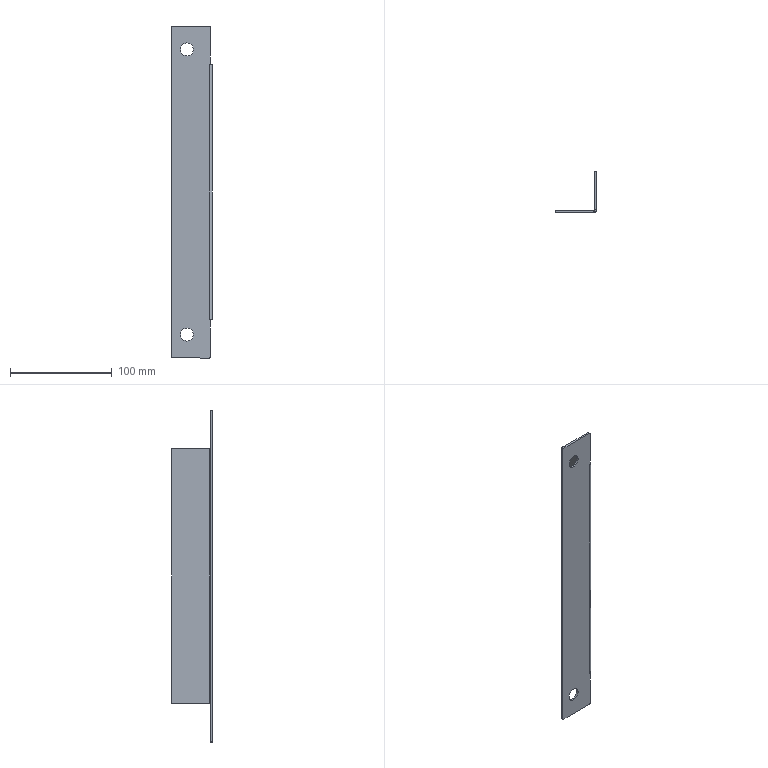Component | SolidWorks | BaseBracketAssembly-1_BaseBracketDepth-9 | 1 solid | 30 faces | box 40 x 40 x 326 mm | volume 43936 mm3 | plane 24 | cylinder 6 | commonest cylinder face diameters 12.639 x4 1 x1 5 x1 | material 2.0mm Cold Rolled Plate
STEP:
#1=COLOUR_RGB('',0.7922,0.8196,0.9333);
#2=FILL_AREA_STYLE_COLOUR('',#1);
#3=FILL_AREA_STYLE('',(#2));
#4=SURFACE_STYLE_FILL_AREA(#3);
#5=SURFACE_SIDE_STYLE('',(#4));
#6=SURFACE_STYLE_USAGE(.BOTH.,#5);
#7=PRESENTATION_STYLE_ASSIGNMENT((#6));
#8=CARTESIAN_POINT('',(9.08,-50.005,25.933));
#9=VERTEX_POINT('',#8);
#10=CARTESIAN_POINT('',(9.08,-50.005,25.436));
#11=VERTEX_POINT('',#10);
#12=CARTESIAN_POINT('',(9.08,-50.005,25.685));
#13=DIRECTION('',(-0.,1.,0.));
#14=DIRECTION('',(-0.,0.,-1.));
#15=AXIS2_PLACEMENT_3D('',#12,#13,#14);
#16=CIRCLE('',#15,0.2488);
#17=EDGE_CURVE('',#9,#11,#16,.T.);
#18=ORIENTED_EDGE('',*,*,#17,.F.);
#19=CARTESIAN_POINT('',(9.08,-49.926,25.933));
#20=VERTEX_POINT('',#19);
#21=CARTESIAN_POINT('',(9.08,-50.32,25.933));
#22=DIRECTION('',(-0.,1.,0.));
#23=VECTOR('',#22,39.37);
#24=LINE('',#21,#23);
#25=EDGE_CURVE('',#9,#20,#24,.T.);
#26=ORIENTED_EDGE('',*,*,#25,.T.);
#27=CARTESIAN_POINT('',(9.08,-49.926,25.436));
#28=VERTEX_POINT('',#27);
#29=CARTESIAN_POINT('',(9.08,-49.926,25.685));
#30=DIRECTION('',(-0.,1.,0.));
#31=DIRECTION('',(-0.,0.,-1.));
#32=AXIS2_PLACEMENT_3D('',#29,#30,#31);
#33=CIRCLE('',#32,0.2488);
#34=EDGE_CURVE('',#20,#28,#33,.T.);
#35=ORIENTED_EDGE('',*,*,#34,.T.);
#36=CARTESIAN_POINT('',(9.08,-50.32,25.436));
#37=DIRECTION('',(-0.,1.,0.));
#38=VECTOR('',#37,39.37);
#39=LINE('',#36,#38);
#40=EDGE_CURVE('',#11,#28,#39,.T.);
#41=ORIENTED_EDGE('',*,*,#40,.F.);
#42=EDGE_LOOP('',(#18,#26,#35,#41));
#43=FACE_OUTER_BOUND('',#42,.T.);
#44=CARTESIAN_POINT('',(9.08,-50.32,25.685));
#45=DIRECTION('',(-0.,1.,0.));
#46=DIRECTION('',(-0.,0.,-1.));
#47=AXIS2_PLACEMENT_3D('',#44,#45,#46);
#48=CYLINDRICAL_SURFACE('',#47,0.2488);
#49=ADVANCED_FACE('',(#43),#48,.F.);
#50=CARTESIAN_POINT('',(9.08,-50.005,36.957));
#51=VERTEX_POINT('',#50);
#52=CARTESIAN_POINT('',(9.08,-50.005,36.459));
#53=VERTEX_POINT('',#52);
#54=CARTESIAN_POINT('',(9.08,-50.005,36.708));
#55=DIRECTION('',(-0.,1.,0.));
#56=DIRECTION('',(-0.,0.,-1.));
#57=AXIS2_PLACEMENT_3D('',#54,#55,#56);
#58=CIRCLE('',#57,0.2488);
#59=EDGE_CURVE('',#51,#53,#58,.T.);
#60=ORIENTED_EDGE('',*,*,#59,.F.);
#61=CARTESIAN_POINT('',(9.08,-49.926,36.957));
#62=VERTEX_POINT('',#61);
#63=CARTESIAN_POINT('',(9.08,-50.32,36.957));
#64=DIRECTION('',(-0.,1.,0.));
#65=VECTOR('',#64,39.37);
#66=LINE('',#63,#65);
#67=EDGE_CURVE('',#51,#62,#66,.T.);
#68=ORIENTED_EDGE('',*,*,#67,.T.);
#69=CARTESIAN_POINT('',(9.08,-49.926,36.459));
#70=VERTEX_POINT('',#69);
#71=CARTESIAN_POINT('',(9.08,-49.926,36.708));
#72=DIRECTION('',(-0.,1.,0.));
#73=DIRECTION('',(-0.,0.,-1.));
#74=AXIS2_PLACEMENT_3D('',#71,#72,#73);
#75=CIRCLE('',#74,0.2488);
#76=EDGE_CURVE('',#62,#70,#75,.T.);
#77=ORIENTED_EDGE('',*,*,#76,.T.);
#78=CARTESIAN_POINT('',(9.08,-50.32,36.459));
#79=DIRECTION('',(-0.,1.,0.));
#80=VECTOR('',#79,39.37);
#81=LINE('',#78,#80);
#82=EDGE_CURVE('',#53,#70,#81,.T.);
#83=ORIENTED_EDGE('',*,*,#82,.F.);
#84=EDGE_LOOP('',(#60,#68,#77,#83));
#85=FACE_OUTER_BOUND('',#84,.T.);
#86=CARTESIAN_POINT('',(9.08,-50.32,36.708));
#87=DIRECTION('',(-0.,1.,0.));
#88=DIRECTION('',(-0.,0.,-1.));
#89=AXIS2_PLACEMENT_3D('',#86,#87,#88);
#90=CYLINDRICAL_SURFACE('',#89,0.2488);
#91=ADVANCED_FACE('',(#85),#90,.F.);
#92=CARTESIAN_POINT('',(9.966,-50.005,26.275));
#93=VERTEX_POINT('',#92);
#94=CARTESIAN_POINT('',(9.962,-50.005,26.275));
#95=VERTEX_POINT('',#94);
#96=CARTESIAN_POINT('',(10.065,-50.005,26.275));
#97=DIRECTION('',(-1.,-0.,0.));
#98=VECTOR('',#97,39.37);
#99=LINE('',#96,#98);
#100=EDGE_CURVE('',#93,#95,#99,.T.);
#101=ORIENTED_EDGE('',*,*,#100,.T.);
#102=CARTESIAN_POINT('',(9.962,-49.926,26.275));
#103=VERTEX_POINT('',#102);
#104=CARTESIAN_POINT('',(9.962,-50.005,26.275));
#105=DIRECTION('',(-0.,1.,0.));
#106=VECTOR('',#105,39.37);
#107=LINE('',#104,#106);
#108=EDGE_CURVE('',#95,#103,#107,.T.);
#109=ORIENTED_EDGE('',*,*,#108,.T.);
#110=CARTESIAN_POINT('',(9.966,-49.926,26.275));
#111=VERTEX_POINT('',#110);
#112=CARTESIAN_POINT('',(10.065,-49.926,26.275));
#113=DIRECTION('',(-1.,-0.,0.));
#114=VECTOR('',#113,39.37);
#115=LINE('',#112,#114);
#116=EDGE_CURVE('',#111,#103,#115,.T.);
#117=ORIENTED_EDGE('',*,*,#116,.F.);
#118=CARTESIAN_POINT('',(9.966,-49.926,26.275));
#119=DIRECTION('',(0.,-1.,-0.));
#120=VECTOR('',#119,39.37);
#121=LINE('',#118,#120);
#122=EDGE_CURVE('',#111,#93,#121,.T.);
#123=ORIENTED_EDGE('',*,*,#122,.T.);
#124=EDGE_LOOP('',(#101,#109,#117,#123));
#125=FACE_OUTER_BOUND('',#124,.T.);
#126=CARTESIAN_POINT('',(9.966,-49.907,26.275));
#127=DIRECTION('',(-0.,0.,-1.));
#128=DIRECTION('',(-1.,-0.,0.));
#129=AXIS2_PLACEMENT_3D('',#126,#127,#128);
#130=PLANE('',#129);
#131=ADVANCED_FACE('',(#125),#130,.T.);
#132=CARTESIAN_POINT('',(10.065,-49.907,26.275));
#133=VERTEX_POINT('',#132);
#134=CARTESIAN_POINT('',(9.986,-49.907,26.275));
#135=VERTEX_POINT('',#134);
#136=CARTESIAN_POINT('',(10.065,-49.907,26.275));
#137=DIRECTION('',(-1.,-0.,0.));
#138=VECTOR('',#137,39.37);
#139=LINE('',#136,#138);
#140=EDGE_CURVE('',#133,#135,#139,.T.);
#141=ORIENTED_EDGE('',*,*,#140,.F.);
#142=CARTESIAN_POINT('',(9.966,-49.907,26.275));
#143=DIRECTION('',(-0.,0.,-1.));
#144=DIRECTION('',(1.,0.,0.));
#145=AXIS2_PLACEMENT_3D('',#142,#143,#144);
#146=CIRCLE('',#145,0.09843);
#147=EDGE_CURVE('',#133,#93,#146,.T.);
#148=ORIENTED_EDGE('',*,*,#147,.T.);
#149=ORIENTED_EDGE('',*,*,#122,.F.);
#150=CARTESIAN_POINT('',(9.966,-49.907,26.275));
#151=DIRECTION('',(-0.,0.,-1.));
#152=DIRECTION('',(-1.,0.,0.));
#153=AXIS2_PLACEMENT_3D('',#150,#151,#152);
#154=CIRCLE('',#153,0.01969);
#155=EDGE_CURVE('',#135,#111,#154,.T.);
#156=ORIENTED_EDGE('',*,*,#155,.F.);
#157=EDGE_LOOP('',(#141,#148,#149,#156));
#158=FACE_OUTER_BOUND('',#157,.T.);
#159=CARTESIAN_POINT('',(10.065,-49.907,26.275));
#160=DIRECTION('',(-0.,0.,-1.));
#161=DIRECTION('',(-1.,-0.,0.));
#162=AXIS2_PLACEMENT_3D('',#159,#160,#161);
#163=PLANE('',#162);
#164=ADVANCED_FACE('',(#158),#163,.T.);
#165=CARTESIAN_POINT('',(10.065,-48.43,26.275));
#166=VERTEX_POINT('',#165);
#167=CARTESIAN_POINT('',(10.065,-48.43,26.275));
#168=DIRECTION('',(0.,-1.,-0.));
#169=VECTOR('',#168,39.37);
#170=LINE('',#167,#169);
#171=EDGE_CURVE('',#166,#133,#170,.T.);
#172=ORIENTED_EDGE('',*,*,#171,.T.);
#173=ORIENTED_EDGE('',*,*,#140,.T.);
#174=CARTESIAN_POINT('',(9.986,-48.43,26.275));
#175=VERTEX_POINT('',#174);
#176=CARTESIAN_POINT('',(9.986,-48.43,26.275));
#177=DIRECTION('',(0.,-1.,-0.));
#178=VECTOR('',#177,39.37);
#179=LINE('',#176,#178);
#180=EDGE_CURVE('',#175,#135,#179,.T.);
#181=ORIENTED_EDGE('',*,*,#180,.F.);
#182=CARTESIAN_POINT('',(10.065,-48.43,26.275));
#183=DIRECTION('',(-1.,-0.,0.));
#184=VECTOR('',#183,39.37);
#185=LINE('',#182,#184);
#186=EDGE_CURVE('',#166,#175,#185,.T.);
#187=ORIENTED_EDGE('',*,*,#186,.F.);
#188=EDGE_LOOP('',(#172,#173,#181,#187));
#189=FACE_OUTER_BOUND('',#188,.T.);
#190=CARTESIAN_POINT('',(9.966,-49.926,26.275));
#191=DIRECTION('',(-0.,0.,-1.));
#192=DIRECTION('',(-1.,-0.,0.));
#193=AXIS2_PLACEMENT_3D('',#190,#191,#192);
#194=PLANE('',#193);
#195=ADVANCED_FACE('',(#189),#194,.T.);
#196=CARTESIAN_POINT('',(9.966,-50.005,36.118));
#197=VERTEX_POINT('',#196);
#198=CARTESIAN_POINT('',(9.966,-49.926,36.118));
#199=VERTEX_POINT('',#198);
#200=CARTESIAN_POINT('',(9.966,-50.005,36.118));
#201=DIRECTION('',(-0.,1.,0.));
#202=VECTOR('',#201,39.37);
#203=LINE('',#200,#202);
#204=EDGE_CURVE('',#197,#199,#203,.T.);
#205=ORIENTED_EDGE('',*,*,#204,.F.);
#206=CARTESIAN_POINT('',(10.065,-49.907,36.118));
#207=VERTEX_POINT('',#206);
#208=CARTESIAN_POINT('',(9.966,-49.907,36.118));
#209=DIRECTION('',(-0.,0.,-1.));
#210=DIRECTION('',(1.,0.,0.));
#211=AXIS2_PLACEMENT_3D('',#208,#209,#210);
#212=CIRCLE('',#211,0.09843);
#213=EDGE_CURVE('',#207,#197,#212,.T.);
#214=ORIENTED_EDGE('',*,*,#213,.F.);
#215=CARTESIAN_POINT('',(9.986,-49.907,36.118));
#216=VERTEX_POINT('',#215);
#217=CARTESIAN_POINT('',(9.986,-49.907,36.118));
#218=DIRECTION('',(1.,0.,-0.));
#219=VECTOR('',#218,39.37);
#220=LINE('',#217,#219);
#221=EDGE_CURVE('',#216,#207,#220,.T.);
#222=ORIENTED_EDGE('',*,*,#221,.F.);
#223=CARTESIAN_POINT('',(9.966,-49.907,36.118));
#224=DIRECTION('',(-0.,0.,-1.));
#225=DIRECTION('',(-1.,0.,0.));
#226=AXIS2_PLACEMENT_3D('',#223,#224,#225);
#227=CIRCLE('',#226,0.01969);
#228=EDGE_CURVE('',#216,#199,#227,.T.);
#229=ORIENTED_EDGE('',*,*,#228,.T.);
#230=EDGE_LOOP('',(#205,#214,#222,#229));
#231=FACE_OUTER_BOUND('',#230,.T.);
#232=CARTESIAN_POINT('',(9.966,-50.005,36.118));
#233=DIRECTION('',(0.,-0.,1.));
#234=DIRECTION('',(1.,0.,-0.));
#235=AXIS2_PLACEMENT_3D('',#232,#233,#234);
#236=PLANE('',#235);
#237=ADVANCED_FACE('',(#231),#236,.T.);
#238=CARTESIAN_POINT('',(9.962,-50.005,36.118));
#239=VERTEX_POINT('',#238);
#240=CARTESIAN_POINT('',(9.962,-49.926,36.118));
#241=VERTEX_POINT('',#240);
#242=CARTESIAN_POINT('',(9.962,-50.005,36.118));
#243=DIRECTION('',(-0.,1.,0.));
#244=VECTOR('',#243,39.37);
#245=LINE('',#242,#244);
#246=EDGE_CURVE('',#239,#241,#245,.T.);
#247=ORIENTED_EDGE('',*,*,#246,.F.);
#248=CARTESIAN_POINT('',(10.065,-50.005,36.118));
#249=DIRECTION('',(-1.,-0.,0.));
#250=VECTOR('',#249,39.37);
#251=LINE('',#248,#250);
#252=EDGE_CURVE('',#197,#239,#251,.T.);
#253=ORIENTED_EDGE('',*,*,#252,.F.);
#254=ORIENTED_EDGE('',*,*,#204,.T.);
#255=CARTESIAN_POINT('',(10.065,-49.926,36.118));
#256=DIRECTION('',(-1.,-0.,0.));
#257=VECTOR('',#256,39.37);
#258=LINE('',#255,#257);
#259=EDGE_CURVE('',#199,#241,#258,.T.);
#260=ORIENTED_EDGE('',*,*,#259,.T.);
#261=EDGE_LOOP('',(#247,#253,#254,#260));
#262=FACE_OUTER_BOUND('',#261,.T.);
#263=CARTESIAN_POINT('',(9.986,-49.907,36.118));
#264=DIRECTION('',(0.,-0.,1.));
#265=DIRECTION('',(1.,0.,-0.));
#266=AXIS2_PLACEMENT_3D('',#263,#264,#265);
#267=PLANE('',#266);
#268=ADVANCED_FACE('',(#262),#267,.T.);
#269=CARTESIAN_POINT('',(9.08,-50.005,25.685));
#270=DIRECTION('',(-0.,1.,0.));
#271=DIRECTION('',(-0.,0.,-1.));
#272=AXIS2_PLACEMENT_3D('',#269,#270,#271);
#273=CIRCLE('',#272,0.2488);
#274=EDGE_CURVE('',#11,#9,#273,.T.);
#275=ORIENTED_EDGE('',*,*,#274,.T.);
#276=ORIENTED_EDGE('',*,*,#17,.T.);
#277=EDGE_LOOP('',(#275,#276));
#278=FACE_BOUND('',#277,.T.);
#279=CARTESIAN_POINT('',(9.08,-50.005,36.708));
#280=DIRECTION('',(-0.,1.,0.));
#281=DIRECTION('',(-0.,0.,-1.));
#282=AXIS2_PLACEMENT_3D('',#279,#280,#281);
#283=CIRCLE('',#282,0.2488);
#284=EDGE_CURVE('',#53,#51,#283,.T.);
#285=ORIENTED_EDGE('',*,*,#284,.T.);
#286=ORIENTED_EDGE('',*,*,#59,.T.);
#287=EDGE_LOOP('',(#285,#286));
#288=FACE_BOUND('',#287,.T.);
#289=CARTESIAN_POINT('',(9.964,-50.005,24.779));
#290=VERTEX_POINT('',#289);
#291=CARTESIAN_POINT('',(9.964,-50.005,24.789));
#292=VERTEX_POINT('',#291);
#293=CARTESIAN_POINT('',(9.964,-50.005,26.275));
#294=DIRECTION('',(0.,-0.,1.));
#295=VECTOR('',#294,39.37);
#296=LINE('',#293,#295);
#297=EDGE_CURVE('',#290,#292,#296,.T.);
#298=ORIENTED_EDGE('',*,*,#297,.T.);
#299=CARTESIAN_POINT('',(9.982,-50.005,24.789));
#300=VERTEX_POINT('',#299);
#301=CARTESIAN_POINT('',(10.065,-50.005,24.789));
#302=DIRECTION('',(1.,0.,-0.));
#303=VECTOR('',#302,39.37);
#304=LINE('',#301,#303);
#305=EDGE_CURVE('',#292,#300,#304,.T.);
#306=ORIENTED_EDGE('',*,*,#305,.T.);
#307=CARTESIAN_POINT('',(9.982,-50.005,26.255));
#308=VERTEX_POINT('',#307);
#309=CARTESIAN_POINT('',(9.982,-50.005,26.255));
#310=DIRECTION('',(0.,-0.,1.));
#311=VECTOR('',#310,39.37);
#312=LINE('',#309,#311);
#313=EDGE_CURVE('',#300,#308,#312,.T.);
#314=ORIENTED_EDGE('',*,*,#313,.T.);
#315=CARTESIAN_POINT('',(9.962,-50.005,26.255));
#316=VERTEX_POINT('',#315);
#317=CARTESIAN_POINT('',(9.982,-50.005,26.255));
#318=DIRECTION('',(-1.,-0.,0.));
#319=VECTOR('',#318,39.37);
#320=LINE('',#317,#319);
#321=EDGE_CURVE('',#308,#316,#320,.T.);
#322=ORIENTED_EDGE('',*,*,#321,.T.);
#323=CARTESIAN_POINT('',(9.962,-50.005,26.275));
#324=DIRECTION('',(0.,-0.,1.));
#325=VECTOR('',#324,39.37);
#326=LINE('',#323,#325);
#327=EDGE_CURVE('',#316,#95,#326,.T.);
#328=ORIENTED_EDGE('',*,*,#327,.T.);
#329=ORIENTED_EDGE('',*,*,#100,.F.);
#330=CARTESIAN_POINT('',(9.966,-50.005,26.275));
#331=DIRECTION('',(0.,-0.,1.));
#332=VECTOR('',#331,39.37);
#333=LINE('',#330,#332);
#334=EDGE_CURVE('',#93,#197,#333,.T.);
#335=ORIENTED_EDGE('',*,*,#334,.T.);
#336=ORIENTED_EDGE('',*,*,#252,.T.);
#337=CARTESIAN_POINT('',(9.962,-50.005,36.137));
#338=VERTEX_POINT('',#337);
#339=CARTESIAN_POINT('',(9.962,-50.005,36.118));
#340=DIRECTION('',(-0.,0.,-1.));
#341=VECTOR('',#340,39.37);
#342=LINE('',#339,#341);
#343=EDGE_CURVE('',#338,#239,#342,.T.);
#344=ORIENTED_EDGE('',*,*,#343,.F.);
#345=CARTESIAN_POINT('',(9.982,-50.005,36.137));
#346=VERTEX_POINT('',#345);
#347=CARTESIAN_POINT('',(9.982,-50.005,36.137));
#348=DIRECTION('',(-1.,-0.,0.));
#349=VECTOR('',#348,39.37);
#350=LINE('',#347,#349);
#351=EDGE_CURVE('',#346,#338,#350,.T.);
#352=ORIENTED_EDGE('',*,*,#351,.F.);
#353=CARTESIAN_POINT('',(9.982,-50.005,37.604));
#354=VERTEX_POINT('',#353);
#355=CARTESIAN_POINT('',(9.982,-50.005,36.137));
#356=DIRECTION('',(-0.,0.,-1.));
#357=VECTOR('',#356,39.37);
#358=LINE('',#355,#357);
#359=EDGE_CURVE('',#354,#346,#358,.T.);
#360=ORIENTED_EDGE('',*,*,#359,.F.);
#361=CARTESIAN_POINT('',(9.964,-50.005,37.604));
#362=VERTEX_POINT('',#361);
#363=CARTESIAN_POINT('',(10.065,-50.005,37.604));
#364=DIRECTION('',(-1.,-0.,0.));
#365=VECTOR('',#364,39.37);
#366=LINE('',#363,#365);
#367=EDGE_CURVE('',#354,#362,#366,.T.);
#368=ORIENTED_EDGE('',*,*,#367,.T.);
#369=CARTESIAN_POINT('',(9.964,-50.005,37.614));
#370=VERTEX_POINT('',#369);
#371=CARTESIAN_POINT('',(9.964,-50.005,26.275));
#372=DIRECTION('',(0.,-0.,1.));
#373=VECTOR('',#372,39.37);
#374=LINE('',#371,#373);
#375=EDGE_CURVE('',#362,#370,#374,.T.);
#376=ORIENTED_EDGE('',*,*,#375,.T.);
#377=CARTESIAN_POINT('',(8.49,-50.005,37.614));
#378=VERTEX_POINT('',#377);
#379=CARTESIAN_POINT('',(8.49,-50.005,37.614));
#380=DIRECTION('',(1.,0.,-0.));
#381=VECTOR('',#380,39.37);
#382=LINE('',#379,#381);
#383=EDGE_CURVE('',#378,#370,#382,.T.);
#384=ORIENTED_EDGE('',*,*,#383,.F.);
#385=CARTESIAN_POINT('',(8.49,-50.005,24.779));
#386=VERTEX_POINT('',#385);
#387=CARTESIAN_POINT('',(8.49,-50.005,26.275));
#388=DIRECTION('',(0.,-0.,1.));
#389=VECTOR('',#388,39.37);
#390=LINE('',#387,#389);
#391=EDGE_CURVE('',#386,#378,#390,.T.);
#392=ORIENTED_EDGE('',*,*,#391,.F.);
#393=CARTESIAN_POINT('',(8.49,-50.005,24.779));
#394=DIRECTION('',(1.,0.,-0.));
#395=VECTOR('',#394,39.37);
#396=LINE('',#393,#395);
#397=EDGE_CURVE('',#386,#290,#396,.T.);
#398=ORIENTED_EDGE('',*,*,#397,.T.);
#399=EDGE_LOOP('',(#298,#306,#314,#322,#328,#329,#335,#336,#344,#352,#360,#368,#376,#384,#392,#398));
#400=FACE_OUTER_BOUND('',#399,.T.);
#401=CARTESIAN_POINT('',(10.065,-50.005,26.275));
#402=DIRECTION('',(-0.,1.,0.));
#403=DIRECTION('',(-0.,0.,-1.));
#404=AXIS2_PLACEMENT_3D('',#401,#402,#403);
#405=PLANE('',#404);
#406=ADVANCED_FACE('',(#278,#288,#400),#405,.F.);
#407=ORIENTED_EDGE('',*,*,#391,.T.);
#408=CARTESIAN_POINT('',(8.49,-49.926,37.614));
#409=VERTEX_POINT('',#408);
#410=CARTESIAN_POINT('',(8.49,-50.005,37.614));
#411=DIRECTION('',(-0.,1.,0.));
#412=VECTOR('',#411,39.37);
#413=LINE('',#410,#412);
#414=EDGE_CURVE('',#378,#409,#413,.T.);
#415=ORIENTED_EDGE('',*,*,#414,.T.);
#416=CARTESIAN_POINT('',(8.49,-49.926,24.779));
#417=VERTEX_POINT('',#416);
#418=CARTESIAN_POINT('',(8.49,-49.926,26.275));
#419=DIRECTION('',(0.,-0.,1.));
#420=VECTOR('',#419,39.37);
#421=LINE('',#418,#420);
#422=EDGE_CURVE('',#417,#409,#421,.T.);
#423=ORIENTED_EDGE('',*,*,#422,.F.);
#424=CARTESIAN_POINT('',(8.49,-50.005,24.779));
#425=DIRECTION('',(-0.,1.,0.));
#426=VECTOR('',#425,39.37);
#427=LINE('',#424,#426);
#428=EDGE_CURVE('',#386,#417,#427,.T.);
#429=ORIENTED_EDGE('',*,*,#428,.F.);
#430=EDGE_LOOP('',(#407,#415,#423,#429));
#431=FACE_OUTER_BOUND('',#430,.T.);
#432=CARTESIAN_POINT('',(8.49,-49.926,26.275));
#433=DIRECTION('',(-1.,-0.,0.));
#434=DIRECTION('',(0.,-0.,1.));
#435=AXIS2_PLACEMENT_3D('',#432,#433,#434);
#436=PLANE('',#435);
#437=ADVANCED_FACE('',(#431),#436,.T.);
#438=CARTESIAN_POINT('',(9.964,-49.926,24.789));
#439=VERTEX_POINT('',#438);
#440=CARTESIAN_POINT('',(9.982,-49.926,24.789));
#441=VERTEX_POINT('',#440);
#442=CARTESIAN_POINT('',(10.065,-49.926,24.789));
#443=DIRECTION('',(1.,0.,-0.));
#444=VECTOR('',#443,39.37);
#445=LINE('',#442,#444);
#446=EDGE_CURVE('',#439,#441,#445,.T.);
#447=ORIENTED_EDGE('',*,*,#446,.F.);
#448=CARTESIAN_POINT('',(9.964,-49.926,24.779));
#449=VERTEX_POINT('',#448);
#450=CARTESIAN_POINT('',(9.964,-49.926,26.275));
#451=DIRECTION('',(0.,-0.,1.));
#452=VECTOR('',#451,39.37);
#453=LINE('',#450,#452);
#454=EDGE_CURVE('',#449,#439,#453,.T.);
#455=ORIENTED_EDGE('',*,*,#454,.F.);
#456=CARTESIAN_POINT('',(8.49,-49.926,24.779));
#457=DIRECTION('',(1.,0.,-0.));
#458=VECTOR('',#457,39.37);
#459=LINE('',#456,#458);
#460=EDGE_CURVE('',#417,#449,#459,.T.);
#461=ORIENTED_EDGE('',*,*,#460,.F.);
#462=ORIENTED_EDGE('',*,*,#422,.T.);
#463=CARTESIAN_POINT('',(9.964,-49.926,37.614));
#464=VERTEX_POINT('',#463);
#465=CARTESIAN_POINT('',(8.49,-49.926,37.614));
#466=DIRECTION('',(1.,0.,-0.));
#467=VECTOR('',#466,39.37);
#468=LINE('',#465,#467);
#469=EDGE_CURVE('',#409,#464,#468,.T.);
#470=ORIENTED_EDGE('',*,*,#469,.T.);
#471=CARTESIAN_POINT('',(9.964,-49.926,37.604));
#472=VERTEX_POINT('',#471);
#473=CARTESIAN_POINT('',(9.964,-49.926,26.275));
#474=DIRECTION('',(0.,-0.,1.));
#475=VECTOR('',#474,39.37);
#476=LINE('',#473,#475);
#477=EDGE_CURVE('',#472,#464,#476,.T.);
#478=ORIENTED_EDGE('',*,*,#477,.F.);
#479=CARTESIAN_POINT('',(9.982,-49.926,37.604));
#480=VERTEX_POINT('',#479);
#481=CARTESIAN_POINT('',(10.065,-49.926,37.604));
#482=DIRECTION('',(-1.,-0.,0.));
#483=VECTOR('',#482,39.37);
#484=LINE('',#481,#483);
#485=EDGE_CURVE('',#480,#472,#484,.T.);
#486=ORIENTED_EDGE('',*,*,#485,.F.);
#487=CARTESIAN_POINT('',(9.982,-49.926,36.137));
#488=VERTEX_POINT('',#487);
#489=CARTESIAN_POINT('',(9.982,-49.926,36.137));
#490=DIRECTION('',(-0.,0.,-1.));
#491=VECTOR('',#490,39.37);
#492=LINE('',#489,#491);
#493=EDGE_CURVE('',#480,#488,#492,.T.);
#494=ORIENTED_EDGE('',*,*,#493,.T.);
#495=CARTESIAN_POINT('',(9.962,-49.926,36.137));
#496=VERTEX_POINT('',#495);
#497=CARTESIAN_POINT('',(9.982,-49.926,36.137));
#498=DIRECTION('',(-1.,-0.,0.));
#499=VECTOR('',#498,39.37);
#500=LINE('',#497,#499);
#501=EDGE_CURVE('',#488,#496,#500,.T.);
#502=ORIENTED_EDGE('',*,*,#501,.T.);
#503=CARTESIAN_POINT('',(9.962,-49.926,36.118));
#504=DIRECTION('',(-0.,0.,-1.));
#505=VECTOR('',#504,39.37);
#506=LINE('',#503,#505);
#507=EDGE_CURVE('',#496,#241,#506,.T.);
#508=ORIENTED_EDGE('',*,*,#507,.T.);
#509=ORIENTED_EDGE('',*,*,#259,.F.);
#510=CARTESIAN_POINT('',(9.966,-49.926,26.275));
#511=DIRECTION('',(0.,-0.,1.));
#512=VECTOR('',#511,39.37);
#513=LINE('',#510,#512);
#514=EDGE_CURVE('',#111,#199,#513,.T.);
#515=ORIENTED_EDGE('',*,*,#514,.F.);
#516=ORIENTED_EDGE('',*,*,#116,.T.);
#517=CARTESIAN_POINT('',(9.962,-49.926,26.255));
#518=VERTEX_POINT('',#517);
#519=CARTESIAN_POINT('',(9.962,-49.926,26.275));
#520=DIRECTION('',(0.,-0.,1.));
#521=VECTOR('',#520,39.37);
#522=LINE('',#519,#521);
#523=EDGE_CURVE('',#518,#103,#522,.T.);
#524=ORIENTED_EDGE('',*,*,#523,.F.);
#525=CARTESIAN_POINT('',(9.982,-49.926,26.255));
#526=VERTEX_POINT('',#525);
#527=CARTESIAN_POINT('',(9.982,-49.926,26.255));
#528=DIRECTION('',(-1.,-0.,0.));
#529=VECTOR('',#528,39.37);
#530=LINE('',#527,#529);
#531=EDGE_CURVE('',#526,#518,#530,.T.);
#532=ORIENTED_EDGE('',*,*,#531,.F.);
#533=CARTESIAN_POINT('',(9.982,-49.926,26.255));
#534=DIRECTION('',(0.,-0.,1.));
#535=VECTOR('',#534,39.37);
#536=LINE('',#533,#535);
#537=EDGE_CURVE('',#441,#526,#536,.T.);
#538=ORIENTED_EDGE('',*,*,#537,.F.);
#539=EDGE_LOOP('',(#447,#455,#461,#462,#470,#478,#486,#494,#502,#508,#509,#515,#516,#524,#532,#538));
#540=FACE_OUTER_BOUND('',#539,.T.);
#541=CARTESIAN_POINT('',(9.08,-49.926,25.685));
#542=DIRECTION('',(-0.,1.,0.));
#543=DIRECTION('',(-0.,0.,-1.));
#544=AXIS2_PLACEMENT_3D('',#541,#542,#543);
#545=CIRCLE('',#544,0.2488);
#546=EDGE_CURVE('',#28,#20,#545,.T.);
#547=ORIENTED_EDGE('',*,*,#546,.F.);
#548=ORIENTED_EDGE('',*,*,#34,.F.);
#549=EDGE_LOOP('',(#547,#548));
#550=FACE_BOUND('',#549,.T.);
#551=CARTESIAN_POINT('',(9.08,-49.926,36.708));
#552=DIRECTION('',(-0.,1.,0.));
#553=DIRECTION('',(-0.,0.,-1.));
#554=AXIS2_PLACEMENT_3D('',#551,#552,#553);
#555=CIRCLE('',#554,0.2488);
#556=EDGE_CURVE('',#70,#62,#555,.T.);
#557=ORIENTED_EDGE('',*,*,#556,.F.);
#558=ORIENTED_EDGE('',*,*,#76,.F.);
#559=EDGE_LOOP('',(#557,#558));
#560=FACE_BOUND('',#559,.T.);
#561=CARTESIAN_POINT('',(10.065,-49.926,26.275));
#562=DIRECTION('',(-0.,1.,0.));
#563=DIRECTION('',(-0.,0.,-1.));
#564=AXIS2_PLACEMENT_3D('',#561,#562,#563);
#565=PLANE('',#564);
#566=ADVANCED_FACE('',(#540,#550,#560),#565,.T.);
#567=ORIENTED_EDGE('',*,*,#228,.F.);
#568=CARTESIAN_POINT('',(9.986,-49.907,26.275));
#569=DIRECTION('',(0.,-0.,1.));
#570=VECTOR('',#569,39.37);
#571=LINE('',#568,#570);
#572=EDGE_CURVE('',#135,#216,#571,.T.);
#573=ORIENTED_EDGE('',*,*,#572,.F.);
#574=ORIENTED_EDGE('',*,*,#155,.T.);
#575=ORIENTED_EDGE('',*,*,#514,.T.);
#576=EDGE_LOOP('',(#567,#573,#574,#575));
#577=FACE_OUTER_BOUND('',#576,.T.);
#578=CARTESIAN_POINT('',(9.966,-49.907,26.275));
#579=DIRECTION('',(0.,-0.,1.));
#580=DIRECTION('',(1.,0.,0.));
#581=AXIS2_PLACEMENT_3D('',#578,#579,#580);
#582=CYLINDRICAL_SURFACE('',#581,0.01969);
#583=ADVANCED_FACE('',(#577),#582,.F.);
#584=CARTESIAN_POINT('',(9.986,-48.43,36.118));
#585=VERTEX_POINT('',#584);
#586=CARTESIAN_POINT('',(9.986,-48.43,36.118));
#587=DIRECTION('',(0.,-1.,-0.));
#588=VECTOR('',#587,39.37);
#589=LINE('',#586,#588);
#590=EDGE_CURVE('',#585,#216,#589,.T.);
#591=ORIENTED_EDGE('',*,*,#590,.F.);
#592=CARTESIAN_POINT('',(9.986,-48.43,26.275));
#593=DIRECTION('',(0.,-0.,1.));
#594=VECTOR('',#593,39.37);
#595=LINE('',#592,#594);
#596=EDGE_CURVE('',#175,#585,#595,.T.);
#597=ORIENTED_EDGE('',*,*,#596,.F.);
#598=ORIENTED_EDGE('',*,*,#180,.T.);
#599=ORIENTED_EDGE('',*,*,#572,.T.);
#600=EDGE_LOOP('',(#591,#597,#598,#599));
#601=FACE_OUTER_BOUND('',#600,.T.);
#602=CARTESIAN_POINT('',(9.986,-48.43,26.275));
#603=DIRECTION('',(-1.,-0.,0.));
#604=DIRECTION('',(-0.,1.,0.));
#605=AXIS2_PLACEMENT_3D('',#602,#603,#604);
#606=PLANE('',#605);
#607=ADVANCED_FACE('',(#601),#606,.T.);
#608=CARTESIAN_POINT('',(10.065,-48.43,36.118));
#609=VERTEX_POINT('',#608);
#610=CARTESIAN_POINT('',(10.065,-48.43,36.118));
#611=DIRECTION('',(-1.,-0.,0.));
#612=VECTOR('',#611,39.37);
#613=LINE('',#610,#612);
#614=EDGE_CURVE('',#609,#585,#613,.T.);
#615=ORIENTED_EDGE('',*,*,#614,.F.);
#616=CARTESIAN_POINT('',(10.065,-48.43,26.275));
#617=DIRECTION('',(0.,-0.,1.));
#618=VECTOR('',#617,39.37);
#619=LINE('',#616,#618);
#620=EDGE_CURVE('',#166,#609,#619,.T.);
#621=ORIENTED_EDGE('',*,*,#620,.F.);
#622=ORIENTED_EDGE('',*,*,#186,.T.);
#623=ORIENTED_EDGE('',*,*,#596,.T.);
#624=EDGE_LOOP('',(#615,#621,#622,#623));
#625=FACE_OUTER_BOUND('',#624,.T.);
#626=CARTESIAN_POINT('',(10.065,-48.43,26.275));
#627=DIRECTION('',(-0.,1.,0.));
#628=DIRECTION('',(1.,0.,-0.));
#629=AXIS2_PLACEMENT_3D('',#626,#627,#628);
#630=PLANE('',#629);
#631=ADVANCED_FACE('',(#625),#630,.T.);
#632=CARTESIAN_POINT('',(10.065,-48.43,36.118));
#633=DIRECTION('',(0.,-1.,-0.));
#634=VECTOR('',#633,39.37);
#635=LINE('',#632,#634);
#636=EDGE_CURVE('',#609,#207,#635,.T.);
#637=ORIENTED_EDGE('',*,*,#636,.T.);
#638=CARTESIAN_POINT('',(10.065,-49.907,26.275));
#639=DIRECTION('',(0.,-0.,1.));
#640=VECTOR('',#639,39.37);
#641=LINE('',#638,#640);
#642=EDGE_CURVE('',#133,#207,#641,.T.);
#643=ORIENTED_EDGE('',*,*,#642,.F.);
#644=ORIENTED_EDGE('',*,*,#171,.F.);
#645=ORIENTED_EDGE('',*,*,#620,.T.);
#646=EDGE_LOOP('',(#637,#643,#644,#645));
#647=FACE_OUTER_BOUND('',#646,.T.);
#648=CARTESIAN_POINT('',(10.065,-48.43,26.275));
#649=DIRECTION('',(-1.,-0.,0.));
#650=DIRECTION('',(-0.,1.,0.));
#651=AXIS2_PLACEMENT_3D('',#648,#649,#650);
#652=PLANE('',#651);
#653=ADVANCED_FACE('',(#647),#652,.F.);
#654=ORIENTED_EDGE('',*,*,#213,.T.);
#655=ORIENTED_EDGE('',*,*,#334,.F.);
#656=ORIENTED_EDGE('',*,*,#147,.F.);
#657=ORIENTED_EDGE('',*,*,#642,.T.);
#658=EDGE_LOOP('',(#654,#655,#656,#657));
#659=FACE_OUTER_BOUND('',#658,.T.);
#660=CARTESIAN_POINT('',(9.966,-49.907,26.275));
#661=DIRECTION('',(0.,-0.,1.));
#662=DIRECTION('',(1.,0.,0.));
#663=AXIS2_PLACEMENT_3D('',#660,#661,#662);
#664=CYLINDRICAL_SURFACE('',#663,0.09843);
#665=ADVANCED_FACE('',(#659),#664,.T.);
#666=ORIENTED_EDGE('',*,*,#590,.T.);
#667=ORIENTED_EDGE('',*,*,#221,.T.);
#668=ORIENTED_EDGE('',*,*,#636,.F.);
#669=ORIENTED_EDGE('',*,*,#614,.T.);
#670=EDGE_LOOP('',(#666,#667,#668,#669));
#671=FACE_OUTER_BOUND('',#670,.T.);
#672=CARTESIAN_POINT('',(9.966,-49.907,36.118));
#673=DIRECTION('',(-0.,0.,-1.));
#674=DIRECTION('',(-1.,-0.,0.));
#675=AXIS2_PLACEMENT_3D('',#672,#673,#674);
#676=PLANE('',#675);
#677=ADVANCED_FACE('',(#671),#676,.F.);
#678=ORIENTED_EDGE('',*,*,#507,.F.);
#679=CARTESIAN_POINT('',(9.962,-50.005,36.137));
#680=DIRECTION('',(-0.,1.,0.));
#681=VECTOR('',#680,39.37);
#682=LINE('',#679,#681);
#683=EDGE_CURVE('',#338,#496,#682,.T.);
#684=ORIENTED_EDGE('',*,*,#683,.F.);
#685=ORIENTED_EDGE('',*,*,#343,.T.);
#686=ORIENTED_EDGE('',*,*,#246,.T.);
#687=EDGE_LOOP('',(#678,#684,#685,#686));
#688=FACE_OUTER_BOUND('',#687,.T.);
#689=CARTESIAN_POINT('',(9.962,-50.005,36.118));
#690=DIRECTION('',(1.,0.,-0.));
#691=DIRECTION('',(-0.,0.,-1.));
#692=AXIS2_PLACEMENT_3D('',#689,#690,#691);
#693=PLANE('',#692);
#694=ADVANCED_FACE('',(#688),#693,.T.);
#695=ORIENTED_EDGE('',*,*,#501,.F.);
#696=CARTESIAN_POINT('',(9.982,-50.005,36.137));
#697=DIRECTION('',(-0.,1.,0.));
#698=VECTOR('',#697,39.37);
#699=LINE('',#696,#698);
#700=EDGE_CURVE('',#346,#488,#699,.T.);
#701=ORIENTED_EDGE('',*,*,#700,.F.);
#702=ORIENTED_EDGE('',*,*,#351,.T.);
#703=ORIENTED_EDGE('',*,*,#683,.T.);
#704=EDGE_LOOP('',(#695,#701,#702,#703));
#705=FACE_OUTER_BOUND('',#704,.T.);
#706=CARTESIAN_POINT('',(9.982,-50.005,36.137));
#707=DIRECTION('',(-0.,0.,-1.));
#708=DIRECTION('',(-1.,-0.,0.));
#709=AXIS2_PLACEMENT_3D('',#706,#707,#708);
#710=PLANE('',#709);
#711=ADVANCED_FACE('',(#705),#710,.T.);
#712=CARTESIAN_POINT('',(9.982,-50.005,37.604));
#713=DIRECTION('',(-0.,1.,0.));
#714=VECTOR('',#713,39.37);
#715=LINE('',#712,#714);
#716=EDGE_CURVE('',#354,#480,#715,.T.);
#717=ORIENTED_EDGE('',*,*,#716,.F.);
#718=ORIENTED_EDGE('',*,*,#359,.T.);
#719=ORIENTED_EDGE('',*,*,#700,.T.);
#720=ORIENTED_EDGE('',*,*,#493,.F.);
#721=EDGE_LOOP('',(#717,#718,#719,#720));
#722=FACE_OUTER_BOUND('',#721,.T.);
#723=CARTESIAN_POINT('',(9.982,-50.005,36.137));
#724=DIRECTION('',(1.,0.,-0.));
#725=DIRECTION('',(-0.,0.,-1.));
#726=AXIS2_PLACEMENT_3D('',#723,#724,#725);
#727=PLANE('',#726);
#728=ADVANCED_FACE('',(#722),#727,.T.);
#729=CARTESIAN_POINT('',(9.964,-50.005,37.614));
#730=DIRECTION('',(0.,-1.,-0.));
#731=VECTOR('',#730,39.37);
#732=LINE('',#729,#731);
#733=EDGE_CURVE('',#464,#370,#732,.T.);
#734=ORIENTED_EDGE('',*,*,#733,.F.);
#735=ORIENTED_EDGE('',*,*,#469,.F.);
#736=ORIENTED_EDGE('',*,*,#414,.F.);
#737=ORIENTED_EDGE('',*,*,#383,.T.);
#738=EDGE_LOOP('',(#734,#735,#736,#737));
#739=FACE_OUTER_BOUND('',#738,.T.);
#740=CARTESIAN_POINT('',(8.49,-50.005,37.614));
#741=DIRECTION('',(0.,-0.,1.));
#742=DIRECTION('',(1.,0.,-0.));
#743=AXIS2_PLACEMENT_3D('',#740,#741,#742);
#744=PLANE('',#743);
#745=ADVANCED_FACE('',(#739),#744,.T.);
#746=ORIENTED_EDGE('',*,*,#460,.T.);
#747=CARTESIAN_POINT('',(9.964,-50.005,24.779));
#748=DIRECTION('',(0.,-1.,-0.));
#749=VECTOR('',#748,39.37);
#750=LINE('',#747,#749);
#751=EDGE_CURVE('',#449,#290,#750,.T.);
#752=ORIENTED_EDGE('',*,*,#751,.T.);
#753=ORIENTED_EDGE('',*,*,#397,.F.);
#754=ORIENTED_EDGE('',*,*,#428,.T.);
#755=EDGE_LOOP('',(#746,#752,#753,#754));
#756=FACE_OUTER_BOUND('',#755,.T.);
#757=CARTESIAN_POINT('',(8.49,-50.005,24.779));
#758=DIRECTION('',(0.,-0.,1.));
#759=DIRECTION('',(1.,0.,-0.));
#760=AXIS2_PLACEMENT_3D('',#757,#758,#759);
#761=PLANE('',#760);
#762=ADVANCED_FACE('',(#756),#761,.F.);
#763=ORIENTED_EDGE('',*,*,#313,.F.);
#764=CARTESIAN_POINT('',(9.982,-50.005,24.789));
#765=DIRECTION('',(-0.,1.,0.));
#766=VECTOR('',#765,39.37);
#767=LINE('',#764,#766);
#768=EDGE_CURVE('',#300,#441,#767,.T.);
#769=ORIENTED_EDGE('',*,*,#768,.T.);
#770=ORIENTED_EDGE('',*,*,#537,.T.);
#771=CARTESIAN_POINT('',(9.982,-50.005,26.255));
#772=DIRECTION('',(-0.,1.,0.));
#773=VECTOR('',#772,39.37);
#774=LINE('',#771,#773);
#775=EDGE_CURVE('',#308,#526,#774,.T.);
#776=ORIENTED_EDGE('',*,*,#775,.F.);
#777=EDGE_LOOP('',(#763,#769,#770,#776));
#778=FACE_OUTER_BOUND('',#777,.T.);
#779=CARTESIAN_POINT('',(9.982,-50.005,26.255));
#780=DIRECTION('',(-1.,-0.,0.));
#781=DIRECTION('',(0.,-0.,1.));
#782=AXIS2_PLACEMENT_3D('',#779,#780,#781);
#783=PLANE('',#782);
#784=ADVANCED_FACE('',(#778),#783,.F.);
#785=ORIENTED_EDGE('',*,*,#531,.T.);
#786=CARTESIAN_POINT('',(9.962,-50.005,26.255));
#787=DIRECTION('',(-0.,1.,0.));
#788=VECTOR('',#787,39.37);
#789=LINE('',#786,#788);
#790=EDGE_CURVE('',#316,#518,#789,.T.);
#791=ORIENTED_EDGE('',*,*,#790,.F.);
#792=ORIENTED_EDGE('',*,*,#321,.F.);
#793=ORIENTED_EDGE('',*,*,#775,.T.);
#794=EDGE_LOOP('',(#785,#791,#792,#793));
#795=FACE_OUTER_BOUND('',#794,.T.);
#796=CARTESIAN_POINT('',(9.982,-50.005,26.255));
#797=DIRECTION('',(-0.,0.,-1.));
#798=DIRECTION('',(-1.,-0.,0.));
#799=AXIS2_PLACEMENT_3D('',#796,#797,#798);
#800=PLANE('',#799);
#801=ADVANCED_FACE('',(#795),#800,.F.);
#802=ORIENTED_EDGE('',*,*,#523,.T.);
#803=ORIENTED_EDGE('',*,*,#108,.F.);
#804=ORIENTED_EDGE('',*,*,#327,.F.);
#805=ORIENTED_EDGE('',*,*,#790,.T.);
#806=EDGE_LOOP('',(#802,#803,#804,#805));
#807=FACE_OUTER_BOUND('',#806,.T.);
#808=CARTESIAN_POINT('',(9.962,-50.005,26.275));
#809=DIRECTION('',(-1.,-0.,0.));
#810=DIRECTION('',(0.,-0.,1.));
#811=AXIS2_PLACEMENT_3D('',#808,#809,#810);
#812=PLANE('',#811);
#813=ADVANCED_FACE('',(#807),#812,.F.);
#814=ORIENTED_EDGE('',*,*,#67,.F.);
#815=ORIENTED_EDGE('',*,*,#284,.F.);
#816=ORIENTED_EDGE('',*,*,#82,.T.);
#817=ORIENTED_EDGE('',*,*,#556,.T.);
#818=EDGE_LOOP('',(#814,#815,#816,#817));
#819=FACE_OUTER_BOUND('',#818,.T.);
#820=CARTESIAN_POINT('',(9.08,-50.32,36.708));
#821=DIRECTION('',(-0.,1.,0.));
#822=DIRECTION('',(-0.,0.,-1.));
#823=AXIS2_PLACEMENT_3D('',#820,#821,#822);
#824=CYLINDRICAL_SURFACE('',#823,0.2488);
#825=ADVANCED_FACE('',(#819),#824,.F.);
#826=ORIENTED_EDGE('',*,*,#25,.F.);
#827=ORIENTED_EDGE('',*,*,#274,.F.);
#828=ORIENTED_EDGE('',*,*,#40,.T.);
#829=ORIENTED_EDGE('',*,*,#546,.T.);
#830=EDGE_LOOP('',(#826,#827,#828,#829));
#831=FACE_OUTER_BOUND('',#830,.T.);
#832=CARTESIAN_POINT('',(9.08,-50.32,25.685));
#833=DIRECTION('',(-0.,1.,0.));
#834=DIRECTION('',(-0.,0.,-1.));
#835=AXIS2_PLACEMENT_3D('',#832,#833,#834);
#836=CYLINDRICAL_SURFACE('',#835,0.2488);
#837=ADVANCED_FACE('',(#831),#836,.F.);
#838=ORIENTED_EDGE('',*,*,#751,.F.);
#839=ORIENTED_EDGE('',*,*,#454,.T.);
#840=CARTESIAN_POINT('',(9.964,-50.013,24.789));
#841=DIRECTION('',(-0.,1.,0.));
#842=VECTOR('',#841,39.37);
#843=LINE('',#840,#842);
#844=EDGE_CURVE('',#292,#439,#843,.T.);
#845=ORIENTED_EDGE('',*,*,#844,.F.);
#846=ORIENTED_EDGE('',*,*,#297,.F.);
#847=EDGE_LOOP('',(#838,#839,#845,#846));
#848=FACE_OUTER_BOUND('',#847,.T.);
#849=CARTESIAN_POINT('',(9.964,-50.013,24.789));
#850=DIRECTION('',(-1.,-0.,0.));
#851=DIRECTION('',(0.,-0.,1.));
#852=AXIS2_PLACEMENT_3D('',#849,#850,#851);
#853=PLANE('',#852);
#854=ADVANCED_FACE('',(#848),#853,.F.);
#855=ORIENTED_EDGE('',*,*,#844,.T.);
#856=ORIENTED_EDGE('',*,*,#446,.T.);
#857=ORIENTED_EDGE('',*,*,#768,.F.);
#858=ORIENTED_EDGE('',*,*,#305,.F.);
#859=EDGE_LOOP('',(#855,#856,#857,#858));
#860=FACE_OUTER_BOUND('',#859,.T.);
#861=CARTESIAN_POINT('',(9.99,-50.013,24.789));
#862=DIRECTION('',(0.,-0.,1.));
#863=DIRECTION('',(1.,0.,-0.));
#864=AXIS2_PLACEMENT_3D('',#861,#862,#863);
#865=PLANE('',#864);
#866=ADVANCED_FACE('',(#860),#865,.F.);
#867=ORIENTED_EDGE('',*,*,#716,.T.);
#868=ORIENTED_EDGE('',*,*,#485,.T.);
#869=CARTESIAN_POINT('',(9.964,-50.013,37.604));
#870=DIRECTION('',(-0.,1.,0.));
#871=VECTOR('',#870,39.37);
#872=LINE('',#869,#871);
#873=EDGE_CURVE('',#362,#472,#872,.T.);
#874=ORIENTED_EDGE('',*,*,#873,.F.);
#875=ORIENTED_EDGE('',*,*,#367,.F.);
#876=EDGE_LOOP('',(#867,#868,#874,#875));
#877=FACE_OUTER_BOUND('',#876,.T.);
#878=CARTESIAN_POINT('',(9.964,-50.013,37.604));
#879=DIRECTION('',(-0.,0.,-1.));
#880=DIRECTION('',(-1.,-0.,0.));
#881=AXIS2_PLACEMENT_3D('',#878,#879,#880);
#882=PLANE('',#881);
#883=ADVANCED_FACE('',(#877),#882,.F.);
#884=ORIENTED_EDGE('',*,*,#873,.T.);
#885=ORIENTED_EDGE('',*,*,#477,.T.);
#886=ORIENTED_EDGE('',*,*,#733,.T.);
#887=ORIENTED_EDGE('',*,*,#375,.F.);
#888=EDGE_LOOP('',(#884,#885,#886,#887));
#889=FACE_OUTER_BOUND('',#888,.T.);
#890=CARTESIAN_POINT('',(9.964,-50.013,37.625));
#891=DIRECTION('',(-1.,-0.,0.));
#892=DIRECTION('',(0.,-0.,1.));
#893=AXIS2_PLACEMENT_3D('',#890,#891,#892);
#894=PLANE('',#893);
#895=ADVANCED_FACE('',(#889),#894,.F.);
#896=CLOSED_SHELL('',(#49,#91,#131,#164,#195,#237,#268,#406,#437,#566,#583,#607,#631,#653,#665,#677,#694,#711,#728,#745,#762,#784,#801,#813,#825,#837,#854,#866,#883,#895));
#897=MANIFOLD_SOLID_BREP('',#896);
#898=STYLED_ITEM('',(#7),#897);
#899=(LENGTH_UNIT()NAMED_UNIT(*)SI_UNIT($,.METRE.));
#900=LENGTH_MEASURE_WITH_UNIT(LENGTH_MEASURE(0.0254),#899);
#901=DIMENSIONAL_EXPONENTS(1.,0.,0.,0.,0.,0.,0.);
#902=(CONVERSION_BASED_UNIT('',#900)LENGTH_UNIT()NAMED_UNIT(#901));
#903=UNCERTAINTY_MEASURE_WITH_UNIT(LENGTH_MEASURE(0.00001),#902,'','');
#904=(NAMED_UNIT(*)PLANE_ANGLE_UNIT()SI_UNIT($,.RADIAN.));
#905=(NAMED_UNIT(*)SI_UNIT($,.STERADIAN.)SOLID_ANGLE_UNIT());
#906=(GEOMETRIC_REPRESENTATION_CONTEXT(3)GLOBAL_UNCERTAINTY_ASSIGNED_CONTEXT((#903))GLOBAL_UNIT_ASSIGNED_CONTEXT((#902,#904,#905))REPRESENTATION_CONTEXT('',''));
#907=MECHANICAL_DESIGN_GEOMETRIC_PRESENTATION_REPRESENTATION('',(#898),#906);
#908=PRESENTATION_LAYER_ASSIGNMENT('','',(#898));
#909=CARTESIAN_POINT('',(0.,0.,0.));
#910=DIRECTION('',(0.,0.,1.));
#911=DIRECTION('',(1.,0.,0.));
#912=AXIS2_PLACEMENT_3D('',#909,#910,#911);
#913=(LENGTH_UNIT()NAMED_UNIT(*)SI_UNIT($,.METRE.));
#914=LENGTH_MEASURE_WITH_UNIT(LENGTH_MEASURE(0.0254),#913);
#915=DIMENSIONAL_EXPONENTS(1.,0.,0.,0.,0.,0.,0.);
#916=(CONVERSION_BASED_UNIT('',#914)LENGTH_UNIT()NAMED_UNIT(#915));
#917=UNCERTAINTY_MEASURE_WITH_UNIT(LENGTH_MEASURE(0.00001),#916,'','');
#918=(NAMED_UNIT(*)PLANE_ANGLE_UNIT()SI_UNIT($,.RADIAN.));
#919=(NAMED_UNIT(*)SI_UNIT($,.STERADIAN.)SOLID_ANGLE_UNIT());
#920=(GEOMETRIC_REPRESENTATION_CONTEXT(3)GLOBAL_UNCERTAINTY_ASSIGNED_CONTEXT((#917))GLOBAL_UNIT_ASSIGNED_CONTEXT((#916,#918,#919))REPRESENTATION_CONTEXT('',''));
#921=ADVANCED_BREP_SHAPE_REPRESENTATION('',(#897,#912),#920);